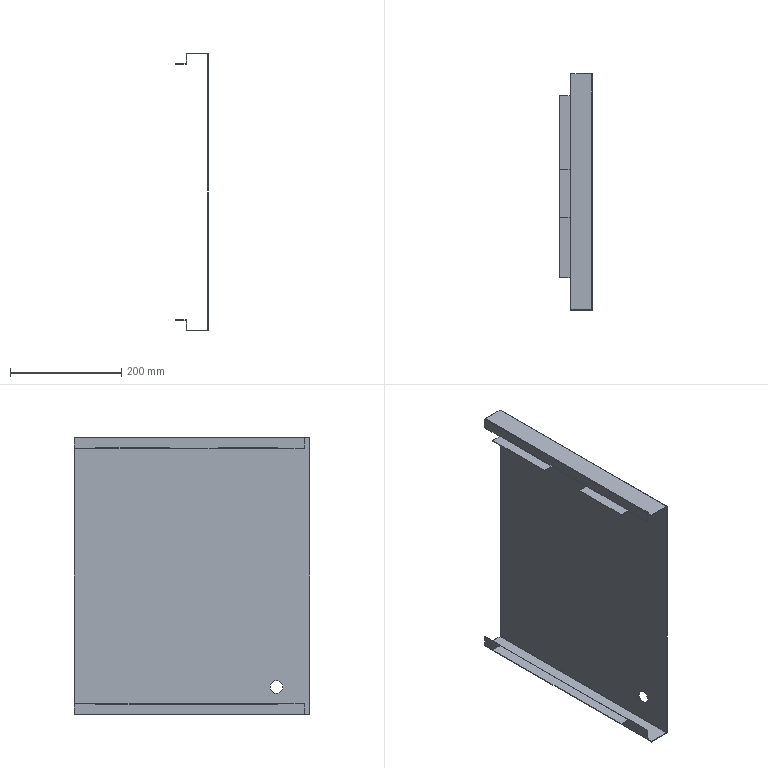Component | SolidWorks | WeldmentDrawing-1_RightSidePanel-1 | 1 solid | 74 faces | volume 323836 mm3 | plane 59 | cylinder 15 | commonest cylinder face diameters 0.2 x7 2.6 x6 23 x2